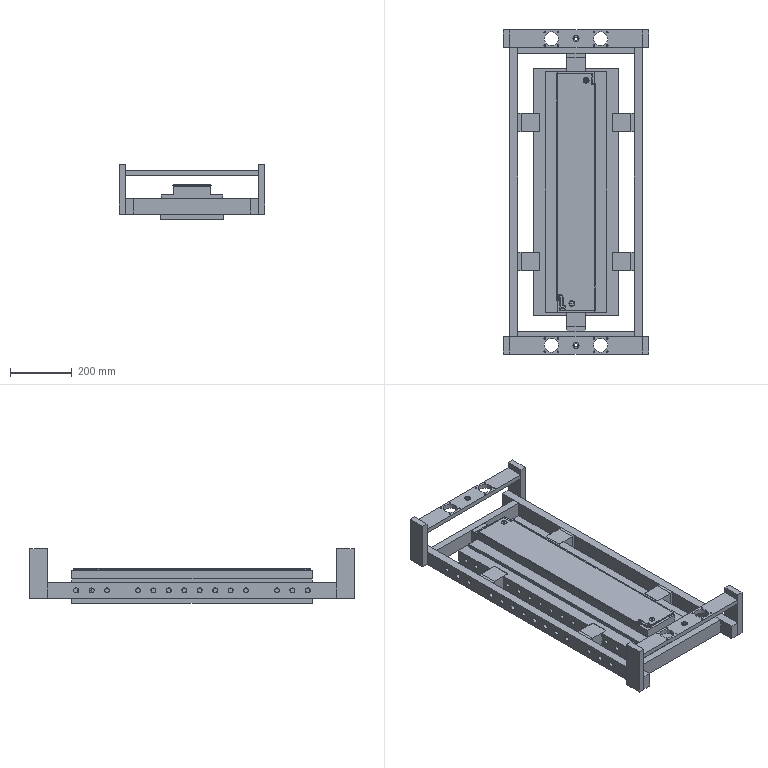Assembly | SolidWorks | mm | 25 component files | 29 solids | 949 faces | box 470 x 1050 x 177 mm | volume 23335690 mm3 | plane 758 | cylinder 181 | cone 7 | spline 3 | commonest cylinder face diameters 5 x32 16 x28 14 x28 4 x20 3.2 x13 7 x12 11 x10 45 x8
Bill of materials:
Cover-glzt-xin.0310 | 1 |  | Long, thin rectangular plate shown as two stacked, slightly offset layers. It has small stepped notches at the ends, small holes and circular markings near the ends, and short tapered bosses or feet on the underside near each end.
Part10 | 2 |  | Solid block extruded from an L-shaped profile: a low base step with a taller upright wall along one side.
Part12 | 1 |  | Rectangular ladder-style frame: two long parallel rails joined by two cross members set in from the rail ends. One rail has a row of small holes along its inner face.
Part18 | 4 |  | Plain rectangular bar or block, taller than it is wide, with a rectangular cross-section.
Part19 | 2 |  | Flat rectangular bar plate with two large round through-holes, each surrounded by four small holes in a square pattern, and one smaller central hole that appears to have a counterbore or recess.
Part37 | 1 |  | Thin, plain rectangular plate.
Part4 | 4 |  | Plain rectangular block or thick plate, wider and taller than it is deep.
Part43 | 1 |  | Stepped plate: a thin rectangular base with a thicker raised section running along its length. The raised top has a long, narrow groove or slot that turns at one end, and there are two small holes near diagonally opposite corners.
Part48 | 2 |  | Plain rectangular block, longer than it is wide or tall.
Part5 | 1 |  | Rectangular plate or slab with small rectangular notches along both long edges and at the middle of each end. There is a row of small round holes along one long side face.
Part51 | 2 |  | Block with an L-shaped profile in plan, with small chamfers on its vertical edges.
Part52 | 4 |  | Block with a C-shaped profile: a rectangular slot is cut in from one side, leaving upper and lower arms. Some vertical edges have small chamfers.
Mates:
1. coincident | Part12-1 face at (127.993, 509, -360) dir (1, 0, 0) | Part18-1 face at (127.993, -512, -330) dir (-1, 0, 0)
2. coincident | Part12-1 face at (-87.007, -16, -410) dir (0, 0, -1) | Part18-1 face at (147.993, -541, -410) dir (0, 0, -1)
3. coincident | Part18-2 face at (-302.007, -512, -330) dir (1, 0, 0) | Part12-1 face at (-302.007, 509, -360) dir (-1, 0, 0)
4. coincident | Part18-2 face at (-302.007, -541, -250) dir (0, -1, 0) | Part12-1 face at (-275.007, -541, -360) dir (0, -1, 0)
5. coincident | Part18-2 face at (-302.007, -541, -410) dir (0, 0, -1) | Part12-1 face at (-87.007, -16, -410) dir (0, 0, -1)
6. coincident | Part18-2 face at (-302.007, -541, -250) dir (0, -1, 0) | Part18-1 face at (147.993, -541, -250) dir (0, -1, 0)
7. coincident | Part12-1 face at (-87.007, -16, -410) dir (0, 0, -1) | Part18-3 face at (-302.007, 451, -410) dir (0, 0, -1)
8. coincident | Part12-1 face at (-275.007, 509, -360) dir (0, 1, 0) | Part18-3 face at (-302.007, 509, -250) dir (0, 1, 0)
9. coincident | Part12-1 face at (-302.007, 509, -360) dir (-1, 0, 0) | Part18-3 face at (-302.007, 480, -330) dir (1, 0, 0)
10. coincident | Part12-1 face at (127.993, 509, -360) dir (1, 0, 0) | Part18-4 face at (127.993, 480, -330) dir (-1, 0, 0)
11. coincident | Part12-1 face at (100.993, 509, -360) dir (0, 1, 0) | Part18-4 face at (147.993, 509, -250) dir (0, 1, 0)
12. coincident | Part12-1 face at (-87.007, -16, -410) dir (0, 0, -1) | Part18-4 face at (147.993, 451, -410) dir (0, 0, -1)
13. distance | Part19-1 face at (-87.007, -512, -270) dir (0, 0, 1) | Part18-2 face at (-302.007, -541, -250) dir (0, 0, 1)
14. coincident | Part18-2 face at (-302.007, -541, -250) dir (0, -1, 0) | Part19-1 face at (-302.007, -541, -270) dir (0, -1, 0)
15. coincident | Part18-2 face at (-302.007, -512, -330) dir (1, 0, 0) | Part19-1 face at (-302.007, -541, -270) dir (-1, 0, 0)
16. coincident | Part18-3 face at (-302.007, 509, -250) dir (0, 1, 0) | Part19-2 face at (-302.007, 509, -270) dir (0, 1, 0)
17. coincident | Part18-3 face at (-302.007, 480, -330) dir (1, 0, 0) | Part19-2 face at (-302.007, 451, -270) dir (-1, 0, 0)
18. distance | Part19-2 face at (-87.007, 480, -270) dir (0, 0, 1) | Part18-3 face at (-302.007, 451, -250) dir (0, 0, 1)
19. coincident | Part12-1 face at (100.993, 509, -360) dir (-1, 0, 0) | Part4-1 face at (100.993, 209, -385) dir (1, 0, 0)
20. coincident | Part12-1 face at (-87.007, -16, -360) dir (0, 0, 1) | Part4-1 face at (100.993, 179, -360) dir (0, 0, 1)
21. coincident | Part12-1 face at (-87.007, -16, -360) dir (0, 0, 1) | Part4-3 face at (100.993, -271, -360) dir (0, 0, 1)
22. coincident | Part12-1 face at (100.993, 509, -360) dir (-1, 0, 0) | Part4-3 face at (100.993, -241, -385) dir (1, 0, 0)
23. coincident | Part12-1 face at (-275.007, 509, -360) dir (1, 0, 0) | Part4-6 face at (-275.007, -241, -385) dir (-1, 0, 0)
24. coincident | Part12-1 face at (-87.007, -16, -360) dir (0, 0, 1) | Part4-6 face at (-265.007, -271, -360) dir (0, 0, 1)
25. coincident | Part12-1 face at (-87.007, -16, -360) dir (0, 0, 1) | Part4-4 face at (-265.007, 179, -360) dir (0, 0, 1)
26. coincident | Part4-1 face at (100.993, 179, -360) dir (0, -1, 0) | Part4-4 face at (-265.007, 179, -360) dir (0, -1, 0)
27. coincident | Part4-3 face at (100.993, -271, -360) dir (0, -1, 0) | Part4-6 face at (-265.007, -271, -360) dir (0, -1, 0)
28. coincident | Part12-1 face at (-87.007, -16, -360) dir (0, 0, 1) | Part5-1 face at (-87.007, -16, -360) dir (0, 0, 1)
29. width | Part5-1 face at (50.493, 384, -360) dir (1, 0, 0) | Part5-1 face at (-224.507, 384, -360) dir (-1, 0, 0) | Part12-1 face at (127.993, 509, -360) dir (1, 0, 0) | Part12-1 face at (-302.007, 509, -360) dir (-1, 0, 0)
30. width | Part5-1 face at (-224.507, 384, -360) dir (0, 1, 0) | Part5-1 face at (-224.507, -416, -360) dir (0, -1, 0) | Part12-1 face at (-275.007, 434, -786.83) dir (0, -1, 0) | Part12-1 face at (-275.007, -466, -786.83) dir (0, 1, 0)
31. coincident | Part12-1 face at (-275.007, 434, -786.83) dir (0, -1, 0) | Part10-1 face at (-117.007, 434, -360) dir (0, 1, 0)
32. coincident | Part12-1 face at (-87.007, -16, -360) dir (0, 0, 1) | Part10-1 face at (-117.007, 419, -360) dir (0, 0, 1)
33. width | Part10-1 face at (-57.007, 434, -410) dir (1, 0, 0) | Part10-1 face at (-117.007, 434, -410) dir (-1, 0, 0) | Part12-1 face at (100.993, 509, -360) dir (-1, 0, 0) | Part12-1 face at (-275.007, 509, -360) dir (1, 0, 0)
34. coincident | Part12-1 face at (-275.007, -466, -786.83) dir (0, 1, 0) | Part10-2 face at (-57.007, -466, -360) dir (0, -1, 0)
35. coincident | Part12-1 face at (-87.007, -16, -360) dir (0, 0, 1) | Part10-2 face at (-57.007, -451, -360) dir (0, 0, 1)
36. coincident | Part10-1 face at (-117.007, 434, -410) dir (-1, 0, 0) | Part10-2 face at (-117.007, -466, -410) dir (-1, 0, 0)
37. coincident | Part5-1 face at (-87.007, -16, -410) dir (0, 0, -1) | Part37-1 face at (-87.007, -16, -410) dir (0, 0, 1)
38. width | Part37-1 face at (15.493, -406, -410) dir (1, 0, 0) | Part37-1 face at (-189.507, -406, -410) dir (-1, 0, 0) | Part5-1 face at (-224.507, 384, -360) dir (-1, 0, 0) | Part5-1 face at (50.493, 384, -360) dir (1, 0, 0)
39. width | Part37-1 face at (15.493, -406, -410) dir (0, -1, 0) | Part37-1 face at (15.493, 374, -410) dir (0, 1, 0) | Part5-1 face at (-224.507, -416, -360) dir (0, -1, 0) | Part5-1 face at (-224.507, 384, -360) dir (0, 1, 0)
40. coincident | Part5-1 face at (-87.007, -16, -360) dir (0, 0, 1) | Part43-1 face at (12.993, -406, -360) dir (0, 0, -1)
41. width | Part43-1 face at (-87.007, -406, -360) dir (0, -1, 0) | Part43-1 face at (-87.007, 374, -360) dir (0, 1, 0) | Part5-1 face at (-224.507, -416, -360) dir (0, -1, 0) | Part5-1 face at (-224.507, 384, -360) dir (0, 1, 0)
42. width | Part43-1 face at (12.993, -406, -360) dir (1, 0, 0) | Part43-1 face at (-187.007, -406, -360) dir (-1, 0, 0) | Part5-1 face at (50.493, 384, -360) dir (1, 0, 0) | Part5-1 face at (-224.507, 384, -360) dir (-1, 0, 0)
43. coincident | Part10-2 face at (-57.007, -421, -395) dir (0, 0, 1) | Part48-1 face at (-87.007, -436, -395) dir (0, 0, -1)
44. coincident | Part10-2 face at (-57.007, -451, -395) dir (0, 1, 0) | Part48-1 face at (-57.007, -451, -385) dir (0, -1, 0)
45. coincident | Part10-2 face at (-117.007, -466, -410) dir (-1, 0, 0) | Part48-1 face at (-117.007, -451, -385) dir (-1, 0, 0)
46. coincident | Part10-1 face at (-117.007, 389, -395) dir (0, 0, 1) | Part48-2 face at (-87.007, 404, -395) dir (0, 0, -1)
47. coincident | Part10-1 face at (-117.007, 419, -395) dir (0, -1, 0) | Part48-2 face at (-57.007, 419, -385) dir (0, 1, 0)
48. coincident | Part10-1 face at (-117.007, 434, -410) dir (-1, 0, 0) | Part48-2 face at (-117.007, 389, -385) dir (-1, 0, 0)
49. coincident | Part5-1 face at (-117.007, 369, -410) dir (0, 1, 0) | Part51-1 face at (-57.007, 369, -360) dir (0, -1, 0)
50. coincident | Part5-1 face at (-87.007, -16, -360) dir (0, 0, 1) | Part51-1 face at (-57.007, 418, -360) dir (0, 0, 1)
51. coincident | Part48-2 face at (-117.007, 389, -385) dir (-1, 0, 0) | Part51-1 face at (-117.007, 369, -360) dir (-1, 0, 0)
52. coincident | Part5-1 face at (-117.007, -401, -410) dir (0, -1, 0) | Part51-2 face at (-117.007, -401, -360) dir (0, 1, 0)
53. coincident | Part5-1 face at (-87.007, -16, -360) dir (0, 0, 1) | Part51-2 face at (-117.007, -450, -360) dir (0, 0, 1)
54. coincident | Part10-2 face at (-117.007, -466, -410) dir (-1, 0, 0) | Part51-2 face at (-117.007, -401, -360) dir (-1, 0, 0)
55. coincident | Part4-4 face at (-265.007, 209, -385) dir (1, 0, 0) | Part52-1 face at (-265.007, 179, -360) dir (-1, 0, 0)
56. coincident | Part5-1 face at (-206.507, 181, -375) dir (0, 0, 1) | Part52-1 face at (-205.007, 179, -375) dir (0, 0, -1)
57. coincident | Part4-1 face at (90.993, 209, -385) dir (-1, 0, 0) | Part52-7 face at (90.993, 179, -410) dir (1, 0, 0)
58. coincident | Part4-1 face at (100.993, 179, -360) dir (0, 0, 1) | Part52-7 face at (90.993, 179, -360) dir (0, 0, 1)
59. coincident | Part4-1 face at (100.993, 239, -360) dir (0, 1, 0) | Part52-7 face at (90.993, 239, -385) dir (0, 1, 0)
60. coincident | Part43-1 face at (-26.007, -406, -320) dir (0, 0, 1) | Cover-glzt-xin.0310-1 face at (-87.007, -16, -320) dir (0, 0, -1)
61. width | Cover-glzt-xin.0310-1 face at (-151.157, 363.1, -318.2) dir (-1, 0, 0) | Cover-glzt-xin.0310-1 face at (-22.857, -395.1, -318.2) dir (1, 0, 0) | Part43-1 face at (-148.007, -406, -348) dir (-1, 0, 0) | Part43-1 face at (-26.007, -406, -348) dir (1, 0, 0)
62. width | Cover-glzt-xin.0310-1 face at (-38.557, 367.9, -318.2) dir (0, 1, 0) | Cover-glzt-xin.0310-1 face at (-27.657, -399.9, -318.2) dir (0, -1, 0) | Part43-1 face at (-87.007, 374, -360) dir (0, 1, 0) | Part43-1 face at (-87.007, -406, -360) dir (0, -1, 0)
63. coincident | Part4-6 face at (-265.007, -241, -385) dir (1, 0, 0) | Part52-6 face at (-265.007, -271, -360) dir (-1, 0, 0)
64. coincident | Part4-6 face at (-265.007, -211, -360) dir (0, 1, 0) | Part52-6 face at (-265.007, -211, -385) dir (0, 1, 0)
65. coincident | Part4-4 face at (-265.007, 239, -360) dir (0, 1, 0) | Part52-1 face at (-265.007, 239, -385) dir (0, 1, 0)
66. coincident | Part5-1 face at (-224.507, 179, -375) dir (0, 1, 0) | Part52-1 face at (-265.007, 179, -385) dir (0, -1, 0)